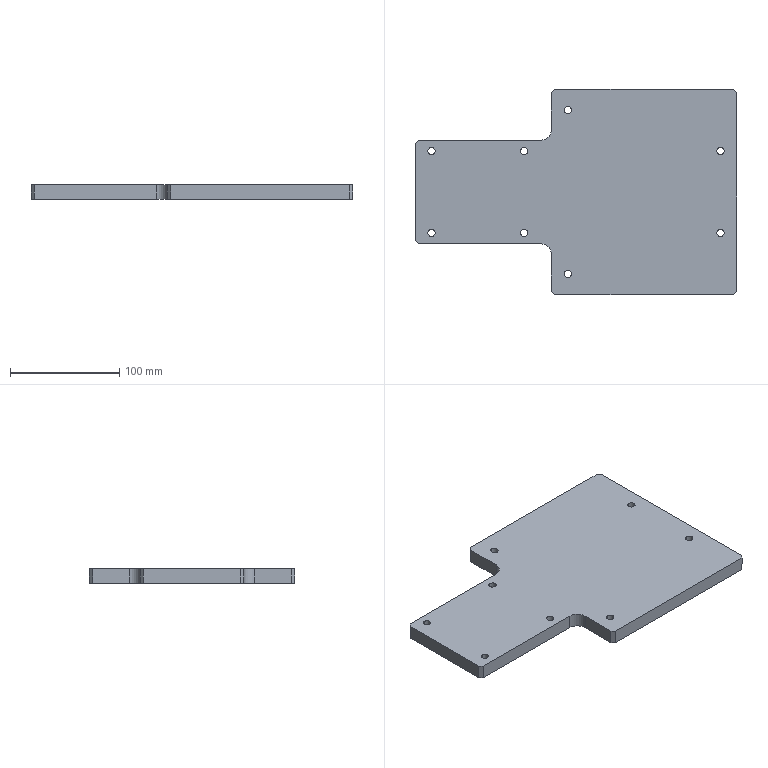Component | SolidWorks | STE21014.01-44-1 | 1 solid | 34 faces | box 295 x 188 x 13 mm | volume 566394 mm3 | cylinder 18 | plane 16 | commonest cylinder face diameters 6.8 x8 6.6 x8 20 x2 | material Q235
STEP:
#1=CARTESIAN_POINT('',(21.457,9.799,-19.331));
#2=VERTEX_POINT('',#1);
#3=CARTESIAN_POINT('',(21.457,9.531,-19.331));
#4=VERTEX_POINT('',#3);
#5=CARTESIAN_POINT('',(21.457,9.665,-19.331));
#6=DIRECTION('',(-0.,-0.,1.));
#7=DIRECTION('',(0.,-1.,0.));
#8=AXIS2_PLACEMENT_3D('',#5,#6,#7);
#9=CIRCLE('',#8,0.1339);
#10=EDGE_CURVE('',#2,#4,#9,.T.);
#11=ORIENTED_EDGE('',*,*,#10,.F.);
#12=CARTESIAN_POINT('',(21.457,9.799,-18.819));
#13=VERTEX_POINT('',#12);
#14=CARTESIAN_POINT('',(21.457,9.799,-18.819));
#15=DIRECTION('',(-0.,-0.,1.));
#16=VECTOR('',#15,39.37);
#17=LINE('',#14,#16);
#18=EDGE_CURVE('',#2,#13,#17,.T.);
#19=ORIENTED_EDGE('',*,*,#18,.T.);
#20=CARTESIAN_POINT('',(21.457,9.531,-18.819));
#21=VERTEX_POINT('',#20);
#22=CARTESIAN_POINT('',(21.457,9.665,-18.819));
#23=DIRECTION('',(-0.,-0.,1.));
#24=DIRECTION('',(0.,-1.,0.));
#25=AXIS2_PLACEMENT_3D('',#22,#23,#24);
#26=CIRCLE('',#25,0.1339);
#27=EDGE_CURVE('',#13,#21,#26,.T.);
#28=ORIENTED_EDGE('',*,*,#27,.T.);
#29=CARTESIAN_POINT('',(21.457,9.531,-18.819));
#30=DIRECTION('',(-0.,-0.,1.));
#31=VECTOR('',#30,39.37);
#32=LINE('',#29,#31);
#33=EDGE_CURVE('',#4,#21,#32,.T.);
#34=ORIENTED_EDGE('',*,*,#33,.F.);
#35=EDGE_LOOP('',(#11,#19,#28,#34));
#36=FACE_OUTER_BOUND('',#35,.T.);
#37=CARTESIAN_POINT('',(21.457,9.665,-18.819));
#38=DIRECTION('',(-0.,-0.,1.));
#39=DIRECTION('',(0.,-1.,0.));
#40=AXIS2_PLACEMENT_3D('',#37,#38,#39);
#41=CYLINDRICAL_SURFACE('',#40,0.1339);
#42=ADVANCED_FACE('',(#36),#41,.F.);
#43=CARTESIAN_POINT('',(21.457,15.705,-19.331));
#44=VERTEX_POINT('',#43);
#45=CARTESIAN_POINT('',(21.457,15.437,-19.331));
#46=VERTEX_POINT('',#45);
#47=CARTESIAN_POINT('',(21.457,15.571,-19.331));
#48=DIRECTION('',(-0.,-0.,1.));
#49=DIRECTION('',(0.,-1.,0.));
#50=AXIS2_PLACEMENT_3D('',#47,#48,#49);
#51=CIRCLE('',#50,0.1339);
#52=EDGE_CURVE('',#44,#46,#51,.T.);
#53=ORIENTED_EDGE('',*,*,#52,.F.);
#54=CARTESIAN_POINT('',(21.457,15.705,-18.819));
#55=VERTEX_POINT('',#54);
#56=CARTESIAN_POINT('',(21.457,15.705,-18.819));
#57=DIRECTION('',(-0.,-0.,1.));
#58=VECTOR('',#57,39.37);
#59=LINE('',#56,#58);
#60=EDGE_CURVE('',#44,#55,#59,.T.);
#61=ORIENTED_EDGE('',*,*,#60,.T.);
#62=CARTESIAN_POINT('',(21.457,15.437,-18.819));
#63=VERTEX_POINT('',#62);
#64=CARTESIAN_POINT('',(21.457,15.571,-18.819));
#65=DIRECTION('',(-0.,-0.,1.));
#66=DIRECTION('',(0.,-1.,0.));
#67=AXIS2_PLACEMENT_3D('',#64,#65,#66);
#68=CIRCLE('',#67,0.1339);
#69=EDGE_CURVE('',#55,#63,#68,.T.);
#70=ORIENTED_EDGE('',*,*,#69,.T.);
#71=CARTESIAN_POINT('',(21.457,15.437,-18.819));
#72=DIRECTION('',(-0.,-0.,1.));
#73=VECTOR('',#72,39.37);
#74=LINE('',#71,#73);
#75=EDGE_CURVE('',#46,#63,#74,.T.);
#76=ORIENTED_EDGE('',*,*,#75,.F.);
#77=EDGE_LOOP('',(#53,#61,#70,#76));
#78=FACE_OUTER_BOUND('',#77,.T.);
#79=CARTESIAN_POINT('',(21.457,15.571,-18.819));
#80=DIRECTION('',(-0.,-0.,1.));
#81=DIRECTION('',(0.,-1.,0.));
#82=AXIS2_PLACEMENT_3D('',#79,#80,#81);
#83=CYLINDRICAL_SURFACE('',#82,0.1339);
#84=ADVANCED_FACE('',(#78),#83,.F.);
#85=CARTESIAN_POINT('',(26.969,14.228,-19.331));
#86=VERTEX_POINT('',#85);
#87=CARTESIAN_POINT('',(26.969,13.961,-19.331));
#88=VERTEX_POINT('',#87);
#89=CARTESIAN_POINT('',(26.969,14.094,-19.331));
#90=DIRECTION('',(-0.,-0.,1.));
#91=DIRECTION('',(0.,-1.,0.));
#92=AXIS2_PLACEMENT_3D('',#89,#90,#91);
#93=CIRCLE('',#92,0.1339);
#94=EDGE_CURVE('',#86,#88,#93,.T.);
#95=ORIENTED_EDGE('',*,*,#94,.F.);
#96=CARTESIAN_POINT('',(26.969,14.228,-18.819));
#97=VERTEX_POINT('',#96);
#98=CARTESIAN_POINT('',(26.969,14.228,-18.819));
#99=DIRECTION('',(-0.,-0.,1.));
#100=VECTOR('',#99,39.37);
#101=LINE('',#98,#100);
#102=EDGE_CURVE('',#86,#97,#101,.T.);
#103=ORIENTED_EDGE('',*,*,#102,.T.);
#104=CARTESIAN_POINT('',(26.969,13.961,-18.819));
#105=VERTEX_POINT('',#104);
#106=CARTESIAN_POINT('',(26.969,14.094,-18.819));
#107=DIRECTION('',(-0.,-0.,1.));
#108=DIRECTION('',(0.,-1.,0.));
#109=AXIS2_PLACEMENT_3D('',#106,#107,#108);
#110=CIRCLE('',#109,0.1339);
#111=EDGE_CURVE('',#97,#105,#110,.T.);
#112=ORIENTED_EDGE('',*,*,#111,.T.);
#113=CARTESIAN_POINT('',(26.969,13.961,-18.819));
#114=DIRECTION('',(-0.,-0.,1.));
#115=VECTOR('',#114,39.37);
#116=LINE('',#113,#115);
#117=EDGE_CURVE('',#88,#105,#116,.T.);
#118=ORIENTED_EDGE('',*,*,#117,.F.);
#119=EDGE_LOOP('',(#95,#103,#112,#118));
#120=FACE_OUTER_BOUND('',#119,.T.);
#121=CARTESIAN_POINT('',(26.969,14.094,-18.819));
#122=DIRECTION('',(-0.,-0.,1.));
#123=DIRECTION('',(0.,-1.,0.));
#124=AXIS2_PLACEMENT_3D('',#121,#122,#123);
#125=CYLINDRICAL_SURFACE('',#124,0.1339);
#126=ADVANCED_FACE('',(#120),#125,.F.);
#127=CARTESIAN_POINT('',(26.969,11.276,-19.331));
#128=VERTEX_POINT('',#127);
#129=CARTESIAN_POINT('',(26.969,11.008,-19.331));
#130=VERTEX_POINT('',#129);
#131=CARTESIAN_POINT('',(26.969,11.142,-19.331));
#132=DIRECTION('',(-0.,-0.,1.));
#133=DIRECTION('',(0.,-1.,0.));
#134=AXIS2_PLACEMENT_3D('',#131,#132,#133);
#135=CIRCLE('',#134,0.1339);
#136=EDGE_CURVE('',#128,#130,#135,.T.);
#137=ORIENTED_EDGE('',*,*,#136,.F.);
#138=CARTESIAN_POINT('',(26.969,11.276,-18.819));
#139=VERTEX_POINT('',#138);
#140=CARTESIAN_POINT('',(26.969,11.276,-18.819));
#141=DIRECTION('',(-0.,-0.,1.));
#142=VECTOR('',#141,39.37);
#143=LINE('',#140,#142);
#144=EDGE_CURVE('',#128,#139,#143,.T.);
#145=ORIENTED_EDGE('',*,*,#144,.T.);
#146=CARTESIAN_POINT('',(26.969,11.008,-18.819));
#147=VERTEX_POINT('',#146);
#148=CARTESIAN_POINT('',(26.969,11.142,-18.819));
#149=DIRECTION('',(-0.,-0.,1.));
#150=DIRECTION('',(0.,-1.,0.));
#151=AXIS2_PLACEMENT_3D('',#148,#149,#150);
#152=CIRCLE('',#151,0.1339);
#153=EDGE_CURVE('',#139,#147,#152,.T.);
#154=ORIENTED_EDGE('',*,*,#153,.T.);
#155=CARTESIAN_POINT('',(26.969,11.008,-18.819));
#156=DIRECTION('',(-0.,-0.,1.));
#157=VECTOR('',#156,39.37);
#158=LINE('',#155,#157);
#159=EDGE_CURVE('',#130,#147,#158,.T.);
#160=ORIENTED_EDGE('',*,*,#159,.F.);
#161=EDGE_LOOP('',(#137,#145,#154,#160));
#162=FACE_OUTER_BOUND('',#161,.T.);
#163=CARTESIAN_POINT('',(26.969,11.142,-18.819));
#164=DIRECTION('',(-0.,-0.,1.));
#165=DIRECTION('',(0.,-1.,0.));
#166=AXIS2_PLACEMENT_3D('',#163,#164,#165);
#167=CYLINDRICAL_SURFACE('',#166,0.1339);
#168=ADVANCED_FACE('',(#162),#167,.F.);
#169=CARTESIAN_POINT('',(16.535,14.224,-19.331));
#170=VERTEX_POINT('',#169);
#171=CARTESIAN_POINT('',(16.535,13.965,-19.331));
#172=VERTEX_POINT('',#171);
#173=CARTESIAN_POINT('',(16.535,14.094,-19.331));
#174=DIRECTION('',(-0.,-0.,1.));
#175=DIRECTION('',(0.,-1.,0.));
#176=AXIS2_PLACEMENT_3D('',#173,#174,#175);
#177=CIRCLE('',#176,0.1299);
#178=EDGE_CURVE('',#170,#172,#177,.T.);
#179=ORIENTED_EDGE('',*,*,#178,.F.);
#180=CARTESIAN_POINT('',(16.535,14.224,-18.819));
#181=VERTEX_POINT('',#180);
#182=CARTESIAN_POINT('',(16.535,14.224,-18.819));
#183=DIRECTION('',(-0.,-0.,1.));
#184=VECTOR('',#183,39.37);
#185=LINE('',#182,#184);
#186=EDGE_CURVE('',#170,#181,#185,.T.);
#187=ORIENTED_EDGE('',*,*,#186,.T.);
#188=CARTESIAN_POINT('',(16.535,13.965,-18.819));
#189=VERTEX_POINT('',#188);
#190=CARTESIAN_POINT('',(16.535,14.094,-18.819));
#191=DIRECTION('',(-0.,-0.,1.));
#192=DIRECTION('',(0.,-1.,0.));
#193=AXIS2_PLACEMENT_3D('',#190,#191,#192);
#194=CIRCLE('',#193,0.1299);
#195=EDGE_CURVE('',#181,#189,#194,.T.);
#196=ORIENTED_EDGE('',*,*,#195,.T.);
#197=CARTESIAN_POINT('',(16.535,13.965,-18.819));
#198=DIRECTION('',(-0.,-0.,1.));
#199=VECTOR('',#198,39.37);
#200=LINE('',#197,#199);
#201=EDGE_CURVE('',#172,#189,#200,.T.);
#202=ORIENTED_EDGE('',*,*,#201,.F.);
#203=EDGE_LOOP('',(#179,#187,#196,#202));
#204=FACE_OUTER_BOUND('',#203,.T.);
#205=CARTESIAN_POINT('',(16.535,14.094,-18.819));
#206=DIRECTION('',(-0.,-0.,1.));
#207=DIRECTION('',(0.,-1.,0.));
#208=AXIS2_PLACEMENT_3D('',#205,#206,#207);
#209=CYLINDRICAL_SURFACE('',#208,0.1299);
#210=ADVANCED_FACE('',(#204),#209,.F.);
#211=CARTESIAN_POINT('',(16.535,11.272,-19.331));
#212=VERTEX_POINT('',#211);
#213=CARTESIAN_POINT('',(16.535,11.012,-19.331));
#214=VERTEX_POINT('',#213);
#215=CARTESIAN_POINT('',(16.535,11.142,-19.331));
#216=DIRECTION('',(-0.,-0.,1.));
#217=DIRECTION('',(0.,-1.,0.));
#218=AXIS2_PLACEMENT_3D('',#215,#216,#217);
#219=CIRCLE('',#218,0.1299);
#220=EDGE_CURVE('',#212,#214,#219,.T.);
#221=ORIENTED_EDGE('',*,*,#220,.F.);
#222=CARTESIAN_POINT('',(16.535,11.272,-18.819));
#223=VERTEX_POINT('',#222);
#224=CARTESIAN_POINT('',(16.535,11.272,-18.819));
#225=DIRECTION('',(-0.,-0.,1.));
#226=VECTOR('',#225,39.37);
#227=LINE('',#224,#226);
#228=EDGE_CURVE('',#212,#223,#227,.T.);
#229=ORIENTED_EDGE('',*,*,#228,.T.);
#230=CARTESIAN_POINT('',(16.535,11.012,-18.819));
#231=VERTEX_POINT('',#230);
#232=CARTESIAN_POINT('',(16.535,11.142,-18.819));
#233=DIRECTION('',(-0.,-0.,1.));
#234=DIRECTION('',(0.,-1.,0.));
#235=AXIS2_PLACEMENT_3D('',#232,#233,#234);
#236=CIRCLE('',#235,0.1299);
#237=EDGE_CURVE('',#223,#231,#236,.T.);
#238=ORIENTED_EDGE('',*,*,#237,.T.);
#239=CARTESIAN_POINT('',(16.535,11.012,-18.819));
#240=DIRECTION('',(-0.,-0.,1.));
#241=VECTOR('',#240,39.37);
#242=LINE('',#239,#241);
#243=EDGE_CURVE('',#214,#231,#242,.T.);
#244=ORIENTED_EDGE('',*,*,#243,.F.);
#245=EDGE_LOOP('',(#221,#229,#238,#244));
#246=FACE_OUTER_BOUND('',#245,.T.);
#247=CARTESIAN_POINT('',(16.535,11.142,-18.819));
#248=DIRECTION('',(-0.,-0.,1.));
#249=DIRECTION('',(0.,-1.,0.));
#250=AXIS2_PLACEMENT_3D('',#247,#248,#249);
#251=CYLINDRICAL_SURFACE('',#250,0.1299);
#252=ADVANCED_FACE('',(#246),#251,.F.);
#253=CARTESIAN_POINT('',(19.882,11.272,-19.331));
#254=VERTEX_POINT('',#253);
#255=CARTESIAN_POINT('',(19.882,11.012,-19.331));
#256=VERTEX_POINT('',#255);
#257=CARTESIAN_POINT('',(19.882,11.142,-19.331));
#258=DIRECTION('',(-0.,-0.,1.));
#259=DIRECTION('',(0.,-1.,0.));
#260=AXIS2_PLACEMENT_3D('',#257,#258,#259);
#261=CIRCLE('',#260,0.1299);
#262=EDGE_CURVE('',#254,#256,#261,.T.);
#263=ORIENTED_EDGE('',*,*,#262,.F.);
#264=CARTESIAN_POINT('',(19.882,11.272,-18.819));
#265=VERTEX_POINT('',#264);
#266=CARTESIAN_POINT('',(19.882,11.272,-18.819));
#267=DIRECTION('',(-0.,-0.,1.));
#268=VECTOR('',#267,39.37);
#269=LINE('',#266,#268);
#270=EDGE_CURVE('',#254,#265,#269,.T.);
#271=ORIENTED_EDGE('',*,*,#270,.T.);
#272=CARTESIAN_POINT('',(19.882,11.012,-18.819));
#273=VERTEX_POINT('',#272);
#274=CARTESIAN_POINT('',(19.882,11.142,-18.819));
#275=DIRECTION('',(-0.,-0.,1.));
#276=DIRECTION('',(0.,-1.,0.));
#277=AXIS2_PLACEMENT_3D('',#274,#275,#276);
#278=CIRCLE('',#277,0.1299);
#279=EDGE_CURVE('',#265,#273,#278,.T.);
#280=ORIENTED_EDGE('',*,*,#279,.T.);
#281=CARTESIAN_POINT('',(19.882,11.012,-18.819));
#282=DIRECTION('',(-0.,-0.,1.));
#283=VECTOR('',#282,39.37);
#284=LINE('',#281,#283);
#285=EDGE_CURVE('',#256,#273,#284,.T.);
#286=ORIENTED_EDGE('',*,*,#285,.F.);
#287=EDGE_LOOP('',(#263,#271,#280,#286));
#288=FACE_OUTER_BOUND('',#287,.T.);
#289=CARTESIAN_POINT('',(19.882,11.142,-18.819));
#290=DIRECTION('',(-0.,-0.,1.));
#291=DIRECTION('',(0.,-1.,0.));
#292=AXIS2_PLACEMENT_3D('',#289,#290,#291);
#293=CYLINDRICAL_SURFACE('',#292,0.1299);
#294=ADVANCED_FACE('',(#288),#293,.F.);
#295=CARTESIAN_POINT('',(19.882,14.224,-19.331));
#296=VERTEX_POINT('',#295);
#297=CARTESIAN_POINT('',(19.882,13.965,-19.331));
#298=VERTEX_POINT('',#297);
#299=CARTESIAN_POINT('',(19.882,14.094,-19.331));
#300=DIRECTION('',(-0.,-0.,1.));
#301=DIRECTION('',(0.,-1.,0.));
#302=AXIS2_PLACEMENT_3D('',#299,#300,#301);
#303=CIRCLE('',#302,0.1299);
#304=EDGE_CURVE('',#296,#298,#303,.T.);
#305=ORIENTED_EDGE('',*,*,#304,.F.);
#306=CARTESIAN_POINT('',(19.882,14.224,-18.819));
#307=VERTEX_POINT('',#306);
#308=CARTESIAN_POINT('',(19.882,14.224,-18.819));
#309=DIRECTION('',(-0.,-0.,1.));
#310=VECTOR('',#309,39.37);
#311=LINE('',#308,#310);
#312=EDGE_CURVE('',#296,#307,#311,.T.);
#313=ORIENTED_EDGE('',*,*,#312,.T.);
#314=CARTESIAN_POINT('',(19.882,13.965,-18.819));
#315=VERTEX_POINT('',#314);
#316=CARTESIAN_POINT('',(19.882,14.094,-18.819));
#317=DIRECTION('',(-0.,-0.,1.));
#318=DIRECTION('',(0.,-1.,0.));
#319=AXIS2_PLACEMENT_3D('',#316,#317,#318);
#320=CIRCLE('',#319,0.1299);
#321=EDGE_CURVE('',#307,#315,#320,.T.);
#322=ORIENTED_EDGE('',*,*,#321,.T.);
#323=CARTESIAN_POINT('',(19.882,13.965,-18.819));
#324=DIRECTION('',(-0.,-0.,1.));
#325=VECTOR('',#324,39.37);
#326=LINE('',#323,#325);
#327=EDGE_CURVE('',#298,#315,#326,.T.);
#328=ORIENTED_EDGE('',*,*,#327,.F.);
#329=EDGE_LOOP('',(#305,#313,#322,#328));
#330=FACE_OUTER_BOUND('',#329,.T.);
#331=CARTESIAN_POINT('',(19.882,14.094,-18.819));
#332=DIRECTION('',(-0.,-0.,1.));
#333=DIRECTION('',(0.,-1.,0.));
#334=AXIS2_PLACEMENT_3D('',#331,#332,#333);
#335=CYLINDRICAL_SURFACE('',#334,0.1299);
#336=ADVANCED_FACE('',(#330),#335,.F.);
#337=CARTESIAN_POINT('',(15.945,14.37,-19.331));
#338=VERTEX_POINT('',#337);
#339=CARTESIAN_POINT('',(15.945,10.866,-19.331));
#340=VERTEX_POINT('',#339);
#341=CARTESIAN_POINT('',(15.945,8.917,-19.331));
#342=DIRECTION('',(0.,-1.,-0.));
#343=VECTOR('',#342,39.37);
#344=LINE('',#341,#343);
#345=EDGE_CURVE('',#338,#340,#344,.T.);
#346=ORIENTED_EDGE('',*,*,#345,.T.);
#347=CARTESIAN_POINT('',(15.945,10.866,-18.819));
#348=VERTEX_POINT('',#347);
#349=CARTESIAN_POINT('',(15.945,10.866,-18.819));
#350=DIRECTION('',(-0.,-0.,1.));
#351=VECTOR('',#350,39.37);
#352=LINE('',#349,#351);
#353=EDGE_CURVE('',#340,#348,#352,.T.);
#354=ORIENTED_EDGE('',*,*,#353,.T.);
#355=CARTESIAN_POINT('',(15.945,14.37,-18.819));
#356=VERTEX_POINT('',#355);
#357=CARTESIAN_POINT('',(15.945,8.917,-18.819));
#358=DIRECTION('',(0.,-1.,-0.));
#359=VECTOR('',#358,39.37);
#360=LINE('',#357,#359);
#361=EDGE_CURVE('',#356,#348,#360,.T.);
#362=ORIENTED_EDGE('',*,*,#361,.F.);
#363=CARTESIAN_POINT('',(15.945,14.37,-18.819));
#364=DIRECTION('',(0.,0.,-1.));
#365=VECTOR('',#364,39.37);
#366=LINE('',#363,#365);
#367=EDGE_CURVE('',#356,#338,#366,.T.);
#368=ORIENTED_EDGE('',*,*,#367,.T.);
#369=EDGE_LOOP('',(#346,#354,#362,#368));
#370=FACE_OUTER_BOUND('',#369,.T.);
#371=CARTESIAN_POINT('',(15.945,8.917,-18.819));
#372=DIRECTION('',(1.,0.,-0.));
#373=DIRECTION('',(-0.,1.,0.));
#374=AXIS2_PLACEMENT_3D('',#371,#372,#373);
#375=PLANE('',#374);
#376=ADVANCED_FACE('',(#370),#375,.F.);
#377=CARTESIAN_POINT('',(20.984,8.917,-18.819));
#378=VERTEX_POINT('',#377);
#379=CARTESIAN_POINT('',(27.441,8.917,-18.819));
#380=VERTEX_POINT('',#379);
#381=CARTESIAN_POINT('',(27.559,8.917,-18.819));
#382=DIRECTION('',(1.,0.,-0.));
#383=VECTOR('',#382,39.37);
#384=LINE('',#381,#383);
#385=EDGE_CURVE('',#378,#380,#384,.T.);
#386=ORIENTED_EDGE('',*,*,#385,.F.);
#387=CARTESIAN_POINT('',(20.984,8.917,-19.331));
#388=VERTEX_POINT('',#387);
#389=CARTESIAN_POINT('',(20.984,8.917,-18.819));
#390=DIRECTION('',(0.,0.,-1.));
#391=VECTOR('',#390,39.37);
#392=LINE('',#389,#391);
#393=EDGE_CURVE('',#378,#388,#392,.T.);
#394=ORIENTED_EDGE('',*,*,#393,.T.);
#395=CARTESIAN_POINT('',(27.441,8.917,-19.331));
#396=VERTEX_POINT('',#395);
#397=CARTESIAN_POINT('',(27.559,8.917,-19.331));
#398=DIRECTION('',(1.,0.,-0.));
#399=VECTOR('',#398,39.37);
#400=LINE('',#397,#399);
#401=EDGE_CURVE('',#388,#396,#400,.T.);
#402=ORIENTED_EDGE('',*,*,#401,.T.);
#403=CARTESIAN_POINT('',(27.441,8.917,-18.819));
#404=DIRECTION('',(-0.,-0.,1.));
#405=VECTOR('',#404,39.37);
#406=LINE('',#403,#405);
#407=EDGE_CURVE('',#396,#380,#406,.T.);
#408=ORIENTED_EDGE('',*,*,#407,.T.);
#409=EDGE_LOOP('',(#386,#394,#402,#408));
#410=FACE_OUTER_BOUND('',#409,.T.);
#411=CARTESIAN_POINT('',(27.559,8.917,-18.819));
#412=DIRECTION('',(-0.,1.,0.));
#413=DIRECTION('',(-1.,-0.,0.));
#414=AXIS2_PLACEMENT_3D('',#411,#412,#413);
#415=PLANE('',#414);
#416=ADVANCED_FACE('',(#410),#415,.F.);
#417=CARTESIAN_POINT('',(27.559,9.035,-18.819));
#418=VERTEX_POINT('',#417);
#419=CARTESIAN_POINT('',(27.559,16.201,-18.819));
#420=VERTEX_POINT('',#419);
#421=CARTESIAN_POINT('',(27.559,8.917,-18.819));
#422=DIRECTION('',(-0.,1.,0.));
#423=VECTOR('',#422,39.37);
#424=LINE('',#421,#423);
#425=EDGE_CURVE('',#418,#420,#424,.T.);
#426=ORIENTED_EDGE('',*,*,#425,.F.);
#427=CARTESIAN_POINT('',(27.559,9.035,-19.331));
#428=VERTEX_POINT('',#427);
#429=CARTESIAN_POINT('',(27.559,9.035,-18.819));
#430=DIRECTION('',(0.,0.,-1.));
#431=VECTOR('',#430,39.37);
#432=LINE('',#429,#431);
#433=EDGE_CURVE('',#418,#428,#432,.T.);
#434=ORIENTED_EDGE('',*,*,#433,.T.);
#435=CARTESIAN_POINT('',(27.559,16.201,-19.331));
#436=VERTEX_POINT('',#435);
#437=CARTESIAN_POINT('',(27.559,8.917,-19.331));
#438=DIRECTION('',(-0.,1.,0.));
#439=VECTOR('',#438,39.37);
#440=LINE('',#437,#439);
#441=EDGE_CURVE('',#428,#436,#440,.T.);
#442=ORIENTED_EDGE('',*,*,#441,.T.);
#443=CARTESIAN_POINT('',(27.559,16.201,-18.819));
#444=DIRECTION('',(-0.,-0.,1.));
#445=VECTOR('',#444,39.37);
#446=LINE('',#443,#445);
#447=EDGE_CURVE('',#436,#420,#446,.T.);
#448=ORIENTED_EDGE('',*,*,#447,.T.);
#449=EDGE_LOOP('',(#426,#434,#442,#448));
#450=FACE_OUTER_BOUND('',#449,.T.);
#451=CARTESIAN_POINT('',(27.559,8.917,-18.819));
#452=DIRECTION('',(-1.,-0.,0.));
#453=DIRECTION('',(0.,-1.,-0.));
#454=AXIS2_PLACEMENT_3D('',#451,#452,#453);
#455=PLANE('',#454);
#456=ADVANCED_FACE('',(#450),#455,.F.);
#457=CARTESIAN_POINT('',(27.441,16.319,-19.331));
#458=VERTEX_POINT('',#457);
#459=CARTESIAN_POINT('',(20.984,16.319,-19.331));
#460=VERTEX_POINT('',#459);
#461=CARTESIAN_POINT('',(27.559,16.319,-19.331));
#462=DIRECTION('',(-1.,-0.,0.));
#463=VECTOR('',#462,39.37);
#464=LINE('',#461,#463);
#465=EDGE_CURVE('',#458,#460,#464,.T.);
#466=ORIENTED_EDGE('',*,*,#465,.T.);
#467=CARTESIAN_POINT('',(20.984,16.319,-18.819));
#468=VERTEX_POINT('',#467);
#469=CARTESIAN_POINT('',(20.984,16.319,-18.819));
#470=DIRECTION('',(-0.,-0.,1.));
#471=VECTOR('',#470,39.37);
#472=LINE('',#469,#471);
#473=EDGE_CURVE('',#460,#468,#472,.T.);
#474=ORIENTED_EDGE('',*,*,#473,.T.);
#475=CARTESIAN_POINT('',(27.441,16.319,-18.819));
#476=VERTEX_POINT('',#475);
#477=CARTESIAN_POINT('',(27.559,16.319,-18.819));
#478=DIRECTION('',(-1.,-0.,0.));
#479=VECTOR('',#478,39.37);
#480=LINE('',#477,#479);
#481=EDGE_CURVE('',#476,#468,#480,.T.);
#482=ORIENTED_EDGE('',*,*,#481,.F.);
#483=CARTESIAN_POINT('',(27.441,16.319,-18.819));
#484=DIRECTION('',(0.,0.,-1.));
#485=VECTOR('',#484,39.37);
#486=LINE('',#483,#485);
#487=EDGE_CURVE('',#476,#458,#486,.T.);
#488=ORIENTED_EDGE('',*,*,#487,.T.);
#489=EDGE_LOOP('',(#466,#474,#482,#488));
#490=FACE_OUTER_BOUND('',#489,.T.);
#491=CARTESIAN_POINT('',(27.559,16.319,-18.819));
#492=DIRECTION('',(0.,-1.,-0.));
#493=DIRECTION('',(1.,0.,-0.));
#494=AXIS2_PLACEMENT_3D('',#491,#492,#493);
#495=PLANE('',#494);
#496=ADVANCED_FACE('',(#490),#495,.F.);
#497=CARTESIAN_POINT('',(21.457,9.665,-18.819));
#498=DIRECTION('',(-0.,-0.,1.));
#499=DIRECTION('',(0.,-1.,0.));
#500=AXIS2_PLACEMENT_3D('',#497,#498,#499);
#501=CIRCLE('',#500,0.1339);
#502=EDGE_CURVE('',#21,#13,#501,.T.);
#503=ORIENTED_EDGE('',*,*,#502,.F.);
#504=ORIENTED_EDGE('',*,*,#27,.F.);
#505=EDGE_LOOP('',(#503,#504));
#506=FACE_BOUND('',#505,.T.);
#507=CARTESIAN_POINT('',(21.457,15.571,-18.819));
#508=DIRECTION('',(-0.,-0.,1.));
#509=DIRECTION('',(0.,-1.,0.));
#510=AXIS2_PLACEMENT_3D('',#507,#508,#509);
#511=CIRCLE('',#510,0.1339);
#512=EDGE_CURVE('',#63,#55,#511,.T.);
#513=ORIENTED_EDGE('',*,*,#512,.F.);
#514=ORIENTED_EDGE('',*,*,#69,.F.);
#515=EDGE_LOOP('',(#513,#514));
#516=FACE_BOUND('',#515,.T.);
#517=CARTESIAN_POINT('',(26.969,14.094,-18.819));
#518=DIRECTION('',(-0.,-0.,1.));
#519=DIRECTION('',(0.,-1.,0.));
#520=AXIS2_PLACEMENT_3D('',#517,#518,#519);
#521=CIRCLE('',#520,0.1339);
#522=EDGE_CURVE('',#105,#97,#521,.T.);
#523=ORIENTED_EDGE('',*,*,#522,.F.);
#524=ORIENTED_EDGE('',*,*,#111,.F.);
#525=EDGE_LOOP('',(#523,#524));
#526=FACE_BOUND('',#525,.T.);
#527=CARTESIAN_POINT('',(26.969,11.142,-18.819));
#528=DIRECTION('',(-0.,-0.,1.));
#529=DIRECTION('',(0.,-1.,0.));
#530=AXIS2_PLACEMENT_3D('',#527,#528,#529);
#531=CIRCLE('',#530,0.1339);
#532=EDGE_CURVE('',#147,#139,#531,.T.);
#533=ORIENTED_EDGE('',*,*,#532,.F.);
#534=ORIENTED_EDGE('',*,*,#153,.F.);
#535=EDGE_LOOP('',(#533,#534));
#536=FACE_BOUND('',#535,.T.);
#537=CARTESIAN_POINT('',(16.535,14.094,-18.819));
#538=DIRECTION('',(-0.,-0.,1.));
#539=DIRECTION('',(0.,-1.,0.));
#540=AXIS2_PLACEMENT_3D('',#537,#538,#539);
#541=CIRCLE('',#540,0.1299);
#542=EDGE_CURVE('',#189,#181,#541,.T.);
#543=ORIENTED_EDGE('',*,*,#542,.F.);
#544=ORIENTED_EDGE('',*,*,#195,.F.);
#545=EDGE_LOOP('',(#543,#544));
#546=FACE_BOUND('',#545,.T.);
#547=CARTESIAN_POINT('',(16.535,11.142,-18.819));
#548=DIRECTION('',(-0.,-0.,1.));
#549=DIRECTION('',(0.,-1.,0.));
#550=AXIS2_PLACEMENT_3D('',#547,#548,#549);
#551=CIRCLE('',#550,0.1299);
#552=EDGE_CURVE('',#231,#223,#551,.T.);
#553=ORIENTED_EDGE('',*,*,#552,.F.);
#554=ORIENTED_EDGE('',*,*,#237,.F.);
#555=EDGE_LOOP('',(#553,#554));
#556=FACE_BOUND('',#555,.T.);
#557=CARTESIAN_POINT('',(19.882,11.142,-18.819));
#558=DIRECTION('',(-0.,-0.,1.));
#559=DIRECTION('',(0.,-1.,0.));
#560=AXIS2_PLACEMENT_3D('',#557,#558,#559);
#561=CIRCLE('',#560,0.1299);
#562=EDGE_CURVE('',#273,#265,#561,.T.);
#563=ORIENTED_EDGE('',*,*,#562,.F.);
#564=ORIENTED_EDGE('',*,*,#279,.F.);
#565=EDGE_LOOP('',(#563,#564));
#566=FACE_BOUND('',#565,.T.);
#567=CARTESIAN_POINT('',(19.882,14.094,-18.819));
#568=DIRECTION('',(-0.,-0.,1.));
#569=DIRECTION('',(0.,-1.,0.));
#570=AXIS2_PLACEMENT_3D('',#567,#568,#569);
#571=CIRCLE('',#570,0.1299);
#572=EDGE_CURVE('',#315,#307,#571,.T.);
#573=ORIENTED_EDGE('',*,*,#572,.F.);
#574=ORIENTED_EDGE('',*,*,#321,.F.);
#575=EDGE_LOOP('',(#573,#574));
#576=FACE_BOUND('',#575,.T.);
#577=ORIENTED_EDGE('',*,*,#361,.T.);
#578=CARTESIAN_POINT('',(16.063,10.748,-18.819));
#579=VERTEX_POINT('',#578);
#580=CARTESIAN_POINT('',(17.972,8.839,-18.819));
#581=DIRECTION('',(0.7071,-0.7071,-0.));
#582=VECTOR('',#581,39.37);
#583=LINE('',#580,#582);
#584=EDGE_CURVE('',#348,#579,#583,.T.);
#585=ORIENTED_EDGE('',*,*,#584,.T.);
#586=CARTESIAN_POINT('',(20.472,10.748,-18.819));
#587=VERTEX_POINT('',#586);
#588=CARTESIAN_POINT('',(15.945,10.748,-18.819));
#589=DIRECTION('',(-1.,-0.,0.));
#590=VECTOR('',#589,39.37);
#591=LINE('',#588,#590);
#592=EDGE_CURVE('',#587,#579,#591,.T.);
#593=ORIENTED_EDGE('',*,*,#592,.F.);
#594=CARTESIAN_POINT('',(20.866,10.354,-18.819));
#595=VERTEX_POINT('',#594);
#596=CARTESIAN_POINT('',(20.472,10.354,-18.819));
#597=DIRECTION('',(0.,0.,-1.));
#598=DIRECTION('',(0.,-1.,0.));
#599=AXIS2_PLACEMENT_3D('',#596,#597,#598);
#600=CIRCLE('',#599,0.3937);
#601=EDGE_CURVE('',#587,#595,#600,.T.);
#602=ORIENTED_EDGE('',*,*,#601,.T.);
#603=CARTESIAN_POINT('',(20.866,9.035,-18.819));
#604=VERTEX_POINT('',#603);
#605=CARTESIAN_POINT('',(20.866,8.917,-18.819));
#606=DIRECTION('',(-0.,1.,0.));
#607=VECTOR('',#606,39.37);
#608=LINE('',#605,#607);
#609=EDGE_CURVE('',#604,#595,#608,.T.);
#610=ORIENTED_EDGE('',*,*,#609,.F.);
#611=CARTESIAN_POINT('',(19.518,10.384,-18.819));
#612=DIRECTION('',(0.7071,-0.7071,-0.));
#613=VECTOR('',#612,39.37);
#614=LINE('',#611,#613);
#615=EDGE_CURVE('',#604,#378,#614,.T.);
#616=ORIENTED_EDGE('',*,*,#615,.T.);
#617=ORIENTED_EDGE('',*,*,#385,.T.);
#618=CARTESIAN_POINT('',(26.447,7.923,-18.819));
#619=DIRECTION('',(0.7071,0.7071,0.));
#620=VECTOR('',#619,39.37);
#621=LINE('',#618,#620);
#622=EDGE_CURVE('',#380,#418,#621,.T.);
#623=ORIENTED_EDGE('',*,*,#622,.T.);
#624=ORIENTED_EDGE('',*,*,#425,.T.);
#625=CARTESIAN_POINT('',(26.447,17.313,-18.819));
#626=DIRECTION('',(-0.7071,0.7071,0.));
#627=VECTOR('',#626,39.37);
#628=LINE('',#625,#627);
#629=EDGE_CURVE('',#420,#476,#628,.T.);
#630=ORIENTED_EDGE('',*,*,#629,.T.);
#631=ORIENTED_EDGE('',*,*,#481,.T.);
#632=CARTESIAN_POINT('',(20.866,16.201,-18.819));
#633=VERTEX_POINT('',#632);
#634=CARTESIAN_POINT('',(19.518,14.852,-18.819));
#635=DIRECTION('',(-0.7071,-0.7071,-0.));
#636=VECTOR('',#635,39.37);
#637=LINE('',#634,#636);
#638=EDGE_CURVE('',#468,#633,#637,.T.);
#639=ORIENTED_EDGE('',*,*,#638,.T.);
#640=CARTESIAN_POINT('',(20.866,14.882,-18.819));
#641=VERTEX_POINT('',#640);
#642=CARTESIAN_POINT('',(20.866,16.319,-18.819));
#643=DIRECTION('',(-0.,1.,0.));
#644=VECTOR('',#643,39.37);
#645=LINE('',#642,#644);
#646=EDGE_CURVE('',#641,#633,#645,.T.);
#647=ORIENTED_EDGE('',*,*,#646,.F.);
#648=CARTESIAN_POINT('',(20.472,14.488,-18.819));
#649=VERTEX_POINT('',#648);
#650=CARTESIAN_POINT('',(20.472,14.882,-18.819));
#651=DIRECTION('',(0.,0.,-1.));
#652=DIRECTION('',(0.,-1.,0.));
#653=AXIS2_PLACEMENT_3D('',#650,#651,#652);
#654=CIRCLE('',#653,0.3937);
#655=EDGE_CURVE('',#641,#649,#654,.T.);
#656=ORIENTED_EDGE('',*,*,#655,.T.);
#657=CARTESIAN_POINT('',(16.063,14.488,-18.819));
#658=VERTEX_POINT('',#657);
#659=CARTESIAN_POINT('',(15.945,14.488,-18.819));
#660=DIRECTION('',(1.,0.,-0.));
#661=VECTOR('',#660,39.37);
#662=LINE('',#659,#661);
#663=EDGE_CURVE('',#658,#649,#662,.T.);
#664=ORIENTED_EDGE('',*,*,#663,.F.);
#665=CARTESIAN_POINT('',(17.972,16.398,-18.819));
#666=DIRECTION('',(-0.7071,-0.7071,-0.));
#667=VECTOR('',#666,39.37);
#668=LINE('',#665,#667);
#669=EDGE_CURVE('',#658,#356,#668,.T.);
#670=ORIENTED_EDGE('',*,*,#669,.T.);
#671=EDGE_LOOP('',(#577,#585,#593,#602,#610,#616,#617,#623,#624,#630,#631,#639,#647,#656,#664,#670));
#672=FACE_OUTER_BOUND('',#671,.T.);
#673=CARTESIAN_POINT('',(21.752,12.618,-18.819));
#674=DIRECTION('',(-0.,-0.,1.));
#675=DIRECTION('',(0.,-1.,-0.));
#676=AXIS2_PLACEMENT_3D('',#673,#674,#675);
#677=PLANE('',#676);
#678=ADVANCED_FACE('',(#506,#516,#526,#536,#546,#556,#566,#576,#672),#677,.T.);
#679=CARTESIAN_POINT('',(21.457,9.665,-19.331));
#680=DIRECTION('',(-0.,-0.,1.));
#681=DIRECTION('',(0.,-1.,0.));
#682=AXIS2_PLACEMENT_3D('',#679,#680,#681);
#683=CIRCLE('',#682,0.1339);
#684=EDGE_CURVE('',#4,#2,#683,.T.);
#685=ORIENTED_EDGE('',*,*,#684,.T.);
#686=ORIENTED_EDGE('',*,*,#10,.T.);
#687=EDGE_LOOP('',(#685,#686));
#688=FACE_BOUND('',#687,.T.);
#689=CARTESIAN_POINT('',(21.457,15.571,-19.331));
#690=DIRECTION('',(-0.,-0.,1.));
#691=DIRECTION('',(0.,-1.,0.));
#692=AXIS2_PLACEMENT_3D('',#689,#690,#691);
#693=CIRCLE('',#692,0.1339);
#694=EDGE_CURVE('',#46,#44,#693,.T.);
#695=ORIENTED_EDGE('',*,*,#694,.T.);
#696=ORIENTED_EDGE('',*,*,#52,.T.);
#697=EDGE_LOOP('',(#695,#696));
#698=FACE_BOUND('',#697,.T.);
#699=CARTESIAN_POINT('',(26.969,14.094,-19.331));
#700=DIRECTION('',(-0.,-0.,1.));
#701=DIRECTION('',(0.,-1.,0.));
#702=AXIS2_PLACEMENT_3D('',#699,#700,#701);
#703=CIRCLE('',#702,0.1339);
#704=EDGE_CURVE('',#88,#86,#703,.T.);
#705=ORIENTED_EDGE('',*,*,#704,.T.);
#706=ORIENTED_EDGE('',*,*,#94,.T.);
#707=EDGE_LOOP('',(#705,#706));
#708=FACE_BOUND('',#707,.T.);
#709=CARTESIAN_POINT('',(26.969,11.142,-19.331));
#710=DIRECTION('',(-0.,-0.,1.));
#711=DIRECTION('',(0.,-1.,0.));
#712=AXIS2_PLACEMENT_3D('',#709,#710,#711);
#713=CIRCLE('',#712,0.1339);
#714=EDGE_CURVE('',#130,#128,#713,.T.);
#715=ORIENTED_EDGE('',*,*,#714,.T.);
#716=ORIENTED_EDGE('',*,*,#136,.T.);
#717=EDGE_LOOP('',(#715,#716));
#718=FACE_BOUND('',#717,.T.);
#719=CARTESIAN_POINT('',(16.535,14.094,-19.331));
#720=DIRECTION('',(-0.,-0.,1.));
#721=DIRECTION('',(0.,-1.,0.));
#722=AXIS2_PLACEMENT_3D('',#719,#720,#721);
#723=CIRCLE('',#722,0.1299);
#724=EDGE_CURVE('',#172,#170,#723,.T.);
#725=ORIENTED_EDGE('',*,*,#724,.T.);
#726=ORIENTED_EDGE('',*,*,#178,.T.);
#727=EDGE_LOOP('',(#725,#726));
#728=FACE_BOUND('',#727,.T.);
#729=CARTESIAN_POINT('',(16.535,11.142,-19.331));
#730=DIRECTION('',(-0.,-0.,1.));
#731=DIRECTION('',(0.,-1.,0.));
#732=AXIS2_PLACEMENT_3D('',#729,#730,#731);
#733=CIRCLE('',#732,0.1299);
#734=EDGE_CURVE('',#214,#212,#733,.T.);
#735=ORIENTED_EDGE('',*,*,#734,.T.);
#736=ORIENTED_EDGE('',*,*,#220,.T.);
#737=EDGE_LOOP('',(#735,#736));
#738=FACE_BOUND('',#737,.T.);
#739=CARTESIAN_POINT('',(19.882,11.142,-19.331));
#740=DIRECTION('',(-0.,-0.,1.));
#741=DIRECTION('',(0.,-1.,0.));
#742=AXIS2_PLACEMENT_3D('',#739,#740,#741);
#743=CIRCLE('',#742,0.1299);
#744=EDGE_CURVE('',#256,#254,#743,.T.);
#745=ORIENTED_EDGE('',*,*,#744,.T.);
#746=ORIENTED_EDGE('',*,*,#262,.T.);
#747=EDGE_LOOP('',(#745,#746));
#748=FACE_BOUND('',#747,.T.);
#749=CARTESIAN_POINT('',(19.882,14.094,-19.331));
#750=DIRECTION('',(-0.,-0.,1.));
#751=DIRECTION('',(0.,-1.,0.));
#752=AXIS2_PLACEMENT_3D('',#749,#750,#751);
#753=CIRCLE('',#752,0.1299);
#754=EDGE_CURVE('',#298,#296,#753,.T.);
#755=ORIENTED_EDGE('',*,*,#754,.T.);
#756=ORIENTED_EDGE('',*,*,#304,.T.);
#757=EDGE_LOOP('',(#755,#756));
#758=FACE_BOUND('',#757,.T.);
#759=CARTESIAN_POINT('',(20.866,9.035,-19.331));
#760=VERTEX_POINT('',#759);
#761=CARTESIAN_POINT('',(20.866,10.354,-19.331));
#762=VERTEX_POINT('',#761);
#763=CARTESIAN_POINT('',(20.866,8.917,-19.331));
#764=DIRECTION('',(-0.,1.,0.));
#765=VECTOR('',#764,39.37);
#766=LINE('',#763,#765);
#767=EDGE_CURVE('',#760,#762,#766,.T.);
#768=ORIENTED_EDGE('',*,*,#767,.T.);
#769=CARTESIAN_POINT('',(20.472,10.748,-19.331));
#770=VERTEX_POINT('',#769);
#771=CARTESIAN_POINT('',(20.472,10.354,-19.331));
#772=DIRECTION('',(-0.,-0.,1.));
#773=DIRECTION('',(0.,-1.,0.));
#774=AXIS2_PLACEMENT_3D('',#771,#772,#773);
#775=CIRCLE('',#774,0.3937);
#776=EDGE_CURVE('',#762,#770,#775,.T.);
#777=ORIENTED_EDGE('',*,*,#776,.T.);
#778=CARTESIAN_POINT('',(16.063,10.748,-19.331));
#779=VERTEX_POINT('',#778);
#780=CARTESIAN_POINT('',(15.945,10.748,-19.331));
#781=DIRECTION('',(-1.,-0.,0.));
#782=VECTOR('',#781,39.37);
#783=LINE('',#780,#782);
#784=EDGE_CURVE('',#770,#779,#783,.T.);
#785=ORIENTED_EDGE('',*,*,#784,.T.);
#786=CARTESIAN_POINT('',(15.945,10.866,-19.331));
#787=DIRECTION('',(-0.7071,0.7071,0.));
#788=VECTOR('',#787,39.37);
#789=LINE('',#786,#788);
#790=EDGE_CURVE('',#779,#340,#789,.T.);
#791=ORIENTED_EDGE('',*,*,#790,.T.);
#792=ORIENTED_EDGE('',*,*,#345,.F.);
#793=CARTESIAN_POINT('',(16.063,14.488,-19.331));
#794=VERTEX_POINT('',#793);
#795=CARTESIAN_POINT('',(16.063,14.488,-19.331));
#796=DIRECTION('',(0.7071,0.7071,0.));
#797=VECTOR('',#796,39.37);
#798=LINE('',#795,#797);
#799=EDGE_CURVE('',#338,#794,#798,.T.);
#800=ORIENTED_EDGE('',*,*,#799,.T.);
#801=CARTESIAN_POINT('',(20.472,14.488,-19.331));
#802=VERTEX_POINT('',#801);
#803=CARTESIAN_POINT('',(15.945,14.488,-19.331));
#804=DIRECTION('',(1.,0.,-0.));
#805=VECTOR('',#804,39.37);
#806=LINE('',#803,#805);
#807=EDGE_CURVE('',#794,#802,#806,.T.);
#808=ORIENTED_EDGE('',*,*,#807,.T.);
#809=CARTESIAN_POINT('',(20.866,14.882,-19.331));
#810=VERTEX_POINT('',#809);
#811=CARTESIAN_POINT('',(20.472,14.882,-19.331));
#812=DIRECTION('',(-0.,-0.,1.));
#813=DIRECTION('',(0.,-1.,0.));
#814=AXIS2_PLACEMENT_3D('',#811,#812,#813);
#815=CIRCLE('',#814,0.3937);
#816=EDGE_CURVE('',#802,#810,#815,.T.);
#817=ORIENTED_EDGE('',*,*,#816,.T.);
#818=CARTESIAN_POINT('',(20.866,16.201,-19.331));
#819=VERTEX_POINT('',#818);
#820=CARTESIAN_POINT('',(20.866,16.319,-19.331));
#821=DIRECTION('',(-0.,1.,0.));
#822=VECTOR('',#821,39.37);
#823=LINE('',#820,#822);
#824=EDGE_CURVE('',#810,#819,#823,.T.);
#825=ORIENTED_EDGE('',*,*,#824,.T.);
#826=CARTESIAN_POINT('',(20.984,16.319,-19.331));
#827=DIRECTION('',(0.7071,0.7071,0.));
#828=VECTOR('',#827,39.37);
#829=LINE('',#826,#828);
#830=EDGE_CURVE('',#819,#460,#829,.T.);
#831=ORIENTED_EDGE('',*,*,#830,.T.);
#832=ORIENTED_EDGE('',*,*,#465,.F.);
#833=CARTESIAN_POINT('',(27.441,16.319,-19.331));
#834=DIRECTION('',(0.7071,-0.7071,-0.));
#835=VECTOR('',#834,39.37);
#836=LINE('',#833,#835);
#837=EDGE_CURVE('',#458,#436,#836,.T.);
#838=ORIENTED_EDGE('',*,*,#837,.T.);
#839=ORIENTED_EDGE('',*,*,#441,.F.);
#840=CARTESIAN_POINT('',(27.559,9.035,-19.331));
#841=DIRECTION('',(-0.7071,-0.7071,-0.));
#842=VECTOR('',#841,39.37);
#843=LINE('',#840,#842);
#844=EDGE_CURVE('',#428,#396,#843,.T.);
#845=ORIENTED_EDGE('',*,*,#844,.T.);
#846=ORIENTED_EDGE('',*,*,#401,.F.);
#847=CARTESIAN_POINT('',(20.866,9.035,-19.331));
#848=DIRECTION('',(-0.7071,0.7071,0.));
#849=VECTOR('',#848,39.37);
#850=LINE('',#847,#849);
#851=EDGE_CURVE('',#388,#760,#850,.T.);
#852=ORIENTED_EDGE('',*,*,#851,.T.);
#853=EDGE_LOOP('',(#768,#777,#785,#791,#792,#800,#808,#817,#825,#831,#832,#838,#839,#845,#846,#852));
#854=FACE_OUTER_BOUND('',#853,.T.);
#855=CARTESIAN_POINT('',(21.752,12.618,-19.331));
#856=DIRECTION('',(-0.,-0.,1.));
#857=DIRECTION('',(0.,-1.,-0.));
#858=AXIS2_PLACEMENT_3D('',#855,#856,#857);
#859=PLANE('',#858);
#860=ADVANCED_FACE('',(#688,#698,#708,#718,#728,#738,#748,#758,#854),#859,.F.);
#861=ORIENTED_EDGE('',*,*,#784,.F.);
#862=CARTESIAN_POINT('',(20.472,10.748,-18.819));
#863=DIRECTION('',(-0.,-0.,1.));
#864=VECTOR('',#863,39.37);
#865=LINE('',#862,#864);
#866=EDGE_CURVE('',#770,#587,#865,.T.);
#867=ORIENTED_EDGE('',*,*,#866,.T.);
#868=ORIENTED_EDGE('',*,*,#592,.T.);
#869=CARTESIAN_POINT('',(16.063,10.748,-19.331));
#870=DIRECTION('',(0.,0.,-1.));
#871=VECTOR('',#870,39.37);
#872=LINE('',#869,#871);
#873=EDGE_CURVE('',#579,#779,#872,.T.);
#874=ORIENTED_EDGE('',*,*,#873,.T.);
#875=EDGE_LOOP('',(#861,#867,#868,#874));
#876=FACE_OUTER_BOUND('',#875,.T.);
#877=CARTESIAN_POINT('',(15.945,10.748,-19.331));
#878=DIRECTION('',(-0.,1.,0.));
#879=DIRECTION('',(-1.,-0.,0.));
#880=AXIS2_PLACEMENT_3D('',#877,#878,#879);
#881=PLANE('',#880);
#882=ADVANCED_FACE('',(#876),#881,.F.);
#883=ORIENTED_EDGE('',*,*,#609,.T.);
#884=CARTESIAN_POINT('',(20.866,10.354,-19.331));
#885=DIRECTION('',(0.,0.,-1.));
#886=VECTOR('',#885,39.37);
#887=LINE('',#884,#886);
#888=EDGE_CURVE('',#595,#762,#887,.T.);
#889=ORIENTED_EDGE('',*,*,#888,.T.);
#890=ORIENTED_EDGE('',*,*,#767,.F.);
#891=CARTESIAN_POINT('',(20.866,9.035,-19.331));
#892=DIRECTION('',(-0.,-0.,1.));
#893=VECTOR('',#892,39.37);
#894=LINE('',#891,#893);
#895=EDGE_CURVE('',#760,#604,#894,.T.);
#896=ORIENTED_EDGE('',*,*,#895,.T.);
#897=EDGE_LOOP('',(#883,#889,#890,#896));
#898=FACE_OUTER_BOUND('',#897,.T.);
#899=CARTESIAN_POINT('',(20.866,8.917,-19.331));
#900=DIRECTION('',(1.,0.,-0.));
#901=DIRECTION('',(-0.,1.,0.));
#902=AXIS2_PLACEMENT_3D('',#899,#900,#901);
#903=PLANE('',#902);
#904=ADVANCED_FACE('',(#898),#903,.F.);
#905=ORIENTED_EDGE('',*,*,#824,.F.);
#906=CARTESIAN_POINT('',(20.866,14.882,-18.819));
#907=DIRECTION('',(-0.,-0.,1.));
#908=VECTOR('',#907,39.37);
#909=LINE('',#906,#908);
#910=EDGE_CURVE('',#810,#641,#909,.T.);
#911=ORIENTED_EDGE('',*,*,#910,.T.);
#912=ORIENTED_EDGE('',*,*,#646,.T.);
#913=CARTESIAN_POINT('',(20.866,16.201,-19.331));
#914=DIRECTION('',(0.,0.,-1.));
#915=VECTOR('',#914,39.37);
#916=LINE('',#913,#915);
#917=EDGE_CURVE('',#633,#819,#916,.T.);
#918=ORIENTED_EDGE('',*,*,#917,.T.);
#919=EDGE_LOOP('',(#905,#911,#912,#918));
#920=FACE_OUTER_BOUND('',#919,.T.);
#921=CARTESIAN_POINT('',(20.866,16.319,-19.331));
#922=DIRECTION('',(1.,0.,-0.));
#923=DIRECTION('',(-0.,1.,0.));
#924=AXIS2_PLACEMENT_3D('',#921,#922,#923);
#925=PLANE('',#924);
#926=ADVANCED_FACE('',(#920),#925,.F.);
#927=ORIENTED_EDGE('',*,*,#663,.T.);
#928=CARTESIAN_POINT('',(20.472,14.488,-19.331));
#929=DIRECTION('',(0.,0.,-1.));
#930=VECTOR('',#929,39.37);
#931=LINE('',#928,#930);
#932=EDGE_CURVE('',#649,#802,#931,.T.);
#933=ORIENTED_EDGE('',*,*,#932,.T.);
#934=ORIENTED_EDGE('',*,*,#807,.F.);
#935=CARTESIAN_POINT('',(16.063,14.488,-19.331));
#936=DIRECTION('',(-0.,-0.,1.));
#937=VECTOR('',#936,39.37);
#938=LINE('',#935,#937);
#939=EDGE_CURVE('',#794,#658,#938,.T.);
#940=ORIENTED_EDGE('',*,*,#939,.T.);
#941=EDGE_LOOP('',(#927,#933,#934,#940));
#942=FACE_OUTER_BOUND('',#941,.T.);
#943=CARTESIAN_POINT('',(15.945,14.488,-19.331));
#944=DIRECTION('',(0.,-1.,-0.));
#945=DIRECTION('',(1.,0.,-0.));
#946=AXIS2_PLACEMENT_3D('',#943,#944,#945);
#947=PLANE('',#946);
#948=ADVANCED_FACE('',(#942),#947,.F.);
#949=ORIENTED_EDGE('',*,*,#312,.F.);
#950=ORIENTED_EDGE('',*,*,#754,.F.);
#951=ORIENTED_EDGE('',*,*,#327,.T.);
#952=ORIENTED_EDGE('',*,*,#572,.T.);
#953=EDGE_LOOP('',(#949,#950,#951,#952));
#954=FACE_OUTER_BOUND('',#953,.T.);
#955=CARTESIAN_POINT('',(19.882,14.094,-18.819));
#956=DIRECTION('',(-0.,-0.,1.));
#957=DIRECTION('',(0.,-1.,0.));
#958=AXIS2_PLACEMENT_3D('',#955,#956,#957);
#959=CYLINDRICAL_SURFACE('',#958,0.1299);
#960=ADVANCED_FACE('',(#954),#959,.F.);
#961=ORIENTED_EDGE('',*,*,#270,.F.);
#962=ORIENTED_EDGE('',*,*,#744,.F.);
#963=ORIENTED_EDGE('',*,*,#285,.T.);
#964=ORIENTED_EDGE('',*,*,#562,.T.);
#965=EDGE_LOOP('',(#961,#962,#963,#964));
#966=FACE_OUTER_BOUND('',#965,.T.);
#967=CARTESIAN_POINT('',(19.882,11.142,-18.819));
#968=DIRECTION('',(-0.,-0.,1.));
#969=DIRECTION('',(0.,-1.,0.));
#970=AXIS2_PLACEMENT_3D('',#967,#968,#969);
#971=CYLINDRICAL_SURFACE('',#970,0.1299);
#972=ADVANCED_FACE('',(#966),#971,.F.);
#973=ORIENTED_EDGE('',*,*,#228,.F.);
#974=ORIENTED_EDGE('',*,*,#734,.F.);
#975=ORIENTED_EDGE('',*,*,#243,.T.);
#976=ORIENTED_EDGE('',*,*,#552,.T.);
#977=EDGE_LOOP('',(#973,#974,#975,#976));
#978=FACE_OUTER_BOUND('',#977,.T.);
#979=CARTESIAN_POINT('',(16.535,11.142,-18.819));
#980=DIRECTION('',(-0.,-0.,1.));
#981=DIRECTION('',(0.,-1.,0.));
#982=AXIS2_PLACEMENT_3D('',#979,#980,#981);
#983=CYLINDRICAL_SURFACE('',#982,0.1299);
#984=ADVANCED_FACE('',(#978),#983,.F.);
#985=ORIENTED_EDGE('',*,*,#186,.F.);
#986=ORIENTED_EDGE('',*,*,#724,.F.);
#987=ORIENTED_EDGE('',*,*,#201,.T.);
#988=ORIENTED_EDGE('',*,*,#542,.T.);
#989=EDGE_LOOP('',(#985,#986,#987,#988));
#990=FACE_OUTER_BOUND('',#989,.T.);
#991=CARTESIAN_POINT('',(16.535,14.094,-18.819));
#992=DIRECTION('',(-0.,-0.,1.));
#993=DIRECTION('',(0.,-1.,0.));
#994=AXIS2_PLACEMENT_3D('',#991,#992,#993);
#995=CYLINDRICAL_SURFACE('',#994,0.1299);
#996=ADVANCED_FACE('',(#990),#995,.F.);
#997=ORIENTED_EDGE('',*,*,#144,.F.);
#998=ORIENTED_EDGE('',*,*,#714,.F.);
#999=ORIENTED_EDGE('',*,*,#159,.T.);
#1000=ORIENTED_EDGE('',*,*,#532,.T.);
#1001=EDGE_LOOP('',(#997,#998,#999,#1000));
#1002=FACE_OUTER_BOUND('',#1001,.T.);
#1003=CARTESIAN_POINT('',(26.969,11.142,-18.819));
#1004=DIRECTION('',(-0.,-0.,1.));
#1005=DIRECTION('',(0.,-1.,0.));
#1006=AXIS2_PLACEMENT_3D('',#1003,#1004,#1005);
#1007=CYLINDRICAL_SURFACE('',#1006,0.1339);
#1008=ADVANCED_FACE('',(#1002),#1007,.F.);
#1009=ORIENTED_EDGE('',*,*,#102,.F.);
#1010=ORIENTED_EDGE('',*,*,#704,.F.);
#1011=ORIENTED_EDGE('',*,*,#117,.T.);
#1012=ORIENTED_EDGE('',*,*,#522,.T.);
#1013=EDGE_LOOP('',(#1009,#1010,#1011,#1012));
#1014=FACE_OUTER_BOUND('',#1013,.T.);
#1015=CARTESIAN_POINT('',(26.969,14.094,-18.819));
#1016=DIRECTION('',(-0.,-0.,1.));
#1017=DIRECTION('',(0.,-1.,0.));
#1018=AXIS2_PLACEMENT_3D('',#1015,#1016,#1017);
#1019=CYLINDRICAL_SURFACE('',#1018,0.1339);
#1020=ADVANCED_FACE('',(#1014),#1019,.F.);
#1021=ORIENTED_EDGE('',*,*,#60,.F.);
#1022=ORIENTED_EDGE('',*,*,#694,.F.);
#1023=ORIENTED_EDGE('',*,*,#75,.T.);
#1024=ORIENTED_EDGE('',*,*,#512,.T.);
#1025=EDGE_LOOP('',(#1021,#1022,#1023,#1024));
#1026=FACE_OUTER_BOUND('',#1025,.T.);
#1027=CARTESIAN_POINT('',(21.457,15.571,-18.819));
#1028=DIRECTION('',(-0.,-0.,1.));
#1029=DIRECTION('',(0.,-1.,0.));
#1030=AXIS2_PLACEMENT_3D('',#1027,#1028,#1029);
#1031=CYLINDRICAL_SURFACE('',#1030,0.1339);
#1032=ADVANCED_FACE('',(#1026),#1031,.F.);
#1033=ORIENTED_EDGE('',*,*,#18,.F.);
#1034=ORIENTED_EDGE('',*,*,#684,.F.);
#1035=ORIENTED_EDGE('',*,*,#33,.T.);
#1036=ORIENTED_EDGE('',*,*,#502,.T.);
#1037=EDGE_LOOP('',(#1033,#1034,#1035,#1036));
#1038=FACE_OUTER_BOUND('',#1037,.T.);
#1039=CARTESIAN_POINT('',(21.457,9.665,-18.819));
#1040=DIRECTION('',(-0.,-0.,1.));
#1041=DIRECTION('',(0.,-1.,0.));
#1042=AXIS2_PLACEMENT_3D('',#1039,#1040,#1041);
#1043=CYLINDRICAL_SURFACE('',#1042,0.1339);
#1044=ADVANCED_FACE('',(#1038),#1043,.F.);
#1045=ORIENTED_EDGE('',*,*,#790,.F.);
#1046=ORIENTED_EDGE('',*,*,#873,.F.);
#1047=ORIENTED_EDGE('',*,*,#584,.F.);
#1048=ORIENTED_EDGE('',*,*,#353,.F.);
#1049=EDGE_LOOP('',(#1045,#1046,#1047,#1048));
#1050=FACE_OUTER_BOUND('',#1049,.T.);
#1051=CARTESIAN_POINT('',(15.945,10.866,-18.819));
#1052=DIRECTION('',(0.7071,0.7071,0.));
#1053=DIRECTION('',(-0.,-0.,1.));
#1054=AXIS2_PLACEMENT_3D('',#1051,#1052,#1053);
#1055=PLANE('',#1054);
#1056=ADVANCED_FACE('',(#1050),#1055,.F.);
#1057=ORIENTED_EDGE('',*,*,#799,.F.);
#1058=ORIENTED_EDGE('',*,*,#367,.F.);
#1059=ORIENTED_EDGE('',*,*,#669,.F.);
#1060=ORIENTED_EDGE('',*,*,#939,.F.);
#1061=EDGE_LOOP('',(#1057,#1058,#1059,#1060));
#1062=FACE_OUTER_BOUND('',#1061,.T.);
#1063=CARTESIAN_POINT('',(16.063,14.488,-19.331));
#1064=DIRECTION('',(0.7071,-0.7071,-0.));
#1065=DIRECTION('',(-0.,-0.,1.));
#1066=AXIS2_PLACEMENT_3D('',#1063,#1064,#1065);
#1067=PLANE('',#1066);
#1068=ADVANCED_FACE('',(#1062),#1067,.F.);
#1069=ORIENTED_EDGE('',*,*,#830,.F.);
#1070=ORIENTED_EDGE('',*,*,#917,.F.);
#1071=ORIENTED_EDGE('',*,*,#638,.F.);
#1072=ORIENTED_EDGE('',*,*,#473,.F.);
#1073=EDGE_LOOP('',(#1069,#1070,#1071,#1072));
#1074=FACE_OUTER_BOUND('',#1073,.T.);
#1075=CARTESIAN_POINT('',(20.984,16.319,-18.819));
#1076=DIRECTION('',(0.7071,-0.7071,-0.));
#1077=DIRECTION('',(-0.,-0.,1.));
#1078=AXIS2_PLACEMENT_3D('',#1075,#1076,#1077);
#1079=PLANE('',#1078);
#1080=ADVANCED_FACE('',(#1074),#1079,.F.);
#1081=ORIENTED_EDGE('',*,*,#851,.F.);
#1082=ORIENTED_EDGE('',*,*,#393,.F.);
#1083=ORIENTED_EDGE('',*,*,#615,.F.);
#1084=ORIENTED_EDGE('',*,*,#895,.F.);
#1085=EDGE_LOOP('',(#1081,#1082,#1083,#1084));
#1086=FACE_OUTER_BOUND('',#1085,.T.);
#1087=CARTESIAN_POINT('',(20.866,9.035,-19.331));
#1088=DIRECTION('',(0.7071,0.7071,0.));
#1089=DIRECTION('',(-0.,-0.,1.));
#1090=AXIS2_PLACEMENT_3D('',#1087,#1088,#1089);
#1091=PLANE('',#1090);
#1092=ADVANCED_FACE('',(#1086),#1091,.F.);
#1093=ORIENTED_EDGE('',*,*,#622,.F.);
#1094=ORIENTED_EDGE('',*,*,#407,.F.);
#1095=ORIENTED_EDGE('',*,*,#844,.F.);
#1096=ORIENTED_EDGE('',*,*,#433,.F.);
#1097=EDGE_LOOP('',(#1093,#1094,#1095,#1096));
#1098=FACE_OUTER_BOUND('',#1097,.T.);
#1099=CARTESIAN_POINT('',(27.559,9.035,-18.819));
#1100=DIRECTION('',(-0.7071,0.7071,0.));
#1101=DIRECTION('',(0.,0.,-1.));
#1102=AXIS2_PLACEMENT_3D('',#1099,#1100,#1101);
#1103=PLANE('',#1102);
#1104=ADVANCED_FACE('',(#1098),#1103,.F.);
#1105=ORIENTED_EDGE('',*,*,#629,.F.);
#1106=ORIENTED_EDGE('',*,*,#447,.F.);
#1107=ORIENTED_EDGE('',*,*,#837,.F.);
#1108=ORIENTED_EDGE('',*,*,#487,.F.);
#1109=EDGE_LOOP('',(#1105,#1106,#1107,#1108));
#1110=FACE_OUTER_BOUND('',#1109,.T.);
#1111=CARTESIAN_POINT('',(27.441,16.319,-18.819));
#1112=DIRECTION('',(-0.7071,-0.7071,-0.));
#1113=DIRECTION('',(0.,0.,-1.));
#1114=AXIS2_PLACEMENT_3D('',#1111,#1112,#1113);
#1115=PLANE('',#1114);
#1116=ADVANCED_FACE('',(#1110),#1115,.F.);
#1117=ORIENTED_EDGE('',*,*,#816,.F.);
#1118=ORIENTED_EDGE('',*,*,#932,.F.);
#1119=ORIENTED_EDGE('',*,*,#655,.F.);
#1120=ORIENTED_EDGE('',*,*,#910,.F.);
#1121=EDGE_LOOP('',(#1117,#1118,#1119,#1120));
#1122=FACE_OUTER_BOUND('',#1121,.T.);
#1123=CARTESIAN_POINT('',(20.472,14.882,-19.331));
#1124=DIRECTION('',(0.,0.,-1.));
#1125=DIRECTION('',(0.,1.,0.));
#1126=AXIS2_PLACEMENT_3D('',#1123,#1124,#1125);
#1127=CYLINDRICAL_SURFACE('',#1126,0.3937);
#1128=ADVANCED_FACE('',(#1122),#1127,.F.);
#1129=ORIENTED_EDGE('',*,*,#776,.F.);
#1130=ORIENTED_EDGE('',*,*,#888,.F.);
#1131=ORIENTED_EDGE('',*,*,#601,.F.);
#1132=ORIENTED_EDGE('',*,*,#866,.F.);
#1133=EDGE_LOOP('',(#1129,#1130,#1131,#1132));
#1134=FACE_OUTER_BOUND('',#1133,.T.);
#1135=CARTESIAN_POINT('',(20.472,10.354,-19.331));
#1136=DIRECTION('',(0.,0.,-1.));
#1137=DIRECTION('',(0.,1.,0.));
#1138=AXIS2_PLACEMENT_3D('',#1135,#1136,#1137);
#1139=CYLINDRICAL_SURFACE('',#1138,0.3937);
#1140=ADVANCED_FACE('',(#1134),#1139,.F.);
#1141=CLOSED_SHELL('',(#42,#84,#126,#168,#210,#252,#294,#336,#376,#416,#456,#496,#678,#860,#882,#904,#926,#948,#960,#972,#984,#996,#1008,#1020,#1032,#1044,#1056,#1068,#1080,#1092,#1104,#1116,#1128,#1140));
#1142=MANIFOLD_SOLID_BREP('',#1141);
#1143=CARTESIAN_POINT('',(0.,0.,0.));
#1144=DIRECTION('',(0.,0.,1.));
#1145=DIRECTION('',(1.,0.,0.));
#1146=AXIS2_PLACEMENT_3D('',#1143,#1144,#1145);
#1147=(LENGTH_UNIT()NAMED_UNIT(*)SI_UNIT($,.METRE.));
#1148=LENGTH_MEASURE_WITH_UNIT(LENGTH_MEASURE(0.0254),#1147);
#1149=DIMENSIONAL_EXPONENTS(1.,0.,0.,0.,0.,0.,0.);
#1150=(CONVERSION_BASED_UNIT('',#1148)LENGTH_UNIT()NAMED_UNIT(#1149));
#1151=UNCERTAINTY_MEASURE_WITH_UNIT(LENGTH_MEASURE(0.00001),#1150,'','');
#1152=(NAMED_UNIT(*)PLANE_ANGLE_UNIT()SI_UNIT($,.RADIAN.));
#1153=(NAMED_UNIT(*)SI_UNIT($,.STERADIAN.)SOLID_ANGLE_UNIT());
#1154=(GEOMETRIC_REPRESENTATION_CONTEXT(3)GLOBAL_UNCERTAINTY_ASSIGNED_CONTEXT((#1151))GLOBAL_UNIT_ASSIGNED_CONTEXT((#1150,#1152,#1153))REPRESENTATION_CONTEXT('',''));
#1155=ADVANCED_BREP_SHAPE_REPRESENTATION('',(#1142,#1146),#1154);
#1156=COLOUR_RGB('',0.7922,0.8196,0.9333);
#1157=FILL_AREA_STYLE_COLOUR('',#1156);
#1158=FILL_AREA_STYLE('',(#1157));
#1159=SURFACE_STYLE_FILL_AREA(#1158);
#1160=SURFACE_SIDE_STYLE('',(#1159));
#1161=SURFACE_STYLE_USAGE(.BOTH.,#1160);
#1162=PRESENTATION_STYLE_ASSIGNMENT((#1161));
#1163=STYLED_ITEM('',(#1162),#1142);
#1164=PRESENTATION_LAYER_ASSIGNMENT('','',(#1163));
#1165=(LENGTH_UNIT()NAMED_UNIT(*)SI_UNIT($,.METRE.));
#1166=LENGTH_MEASURE_WITH_UNIT(LENGTH_MEASURE(0.0254),#1165);
#1167=DIMENSIONAL_EXPONENTS(1.,0.,0.,0.,0.,0.,0.);
#1168=(CONVERSION_BASED_UNIT('',#1166)LENGTH_UNIT()NAMED_UNIT(#1167));
#1169=UNCERTAINTY_MEASURE_WITH_UNIT(LENGTH_MEASURE(0.00001),#1168,'','');
#1170=(NAMED_UNIT(*)PLANE_ANGLE_UNIT()SI_UNIT($,.RADIAN.));
#1171=(NAMED_UNIT(*)SI_UNIT($,.STERADIAN.)SOLID_ANGLE_UNIT());
#1172=(GEOMETRIC_REPRESENTATION_CONTEXT(3)GLOBAL_UNCERTAINTY_ASSIGNED_CONTEXT((#1169))GLOBAL_UNIT_ASSIGNED_CONTEXT((#1168,#1170,#1171))REPRESENTATION_CONTEXT('',''));
#1173=MECHANICAL_DESIGN_GEOMETRIC_PRESENTATION_REPRESENTATION('',(#1163),#1172);